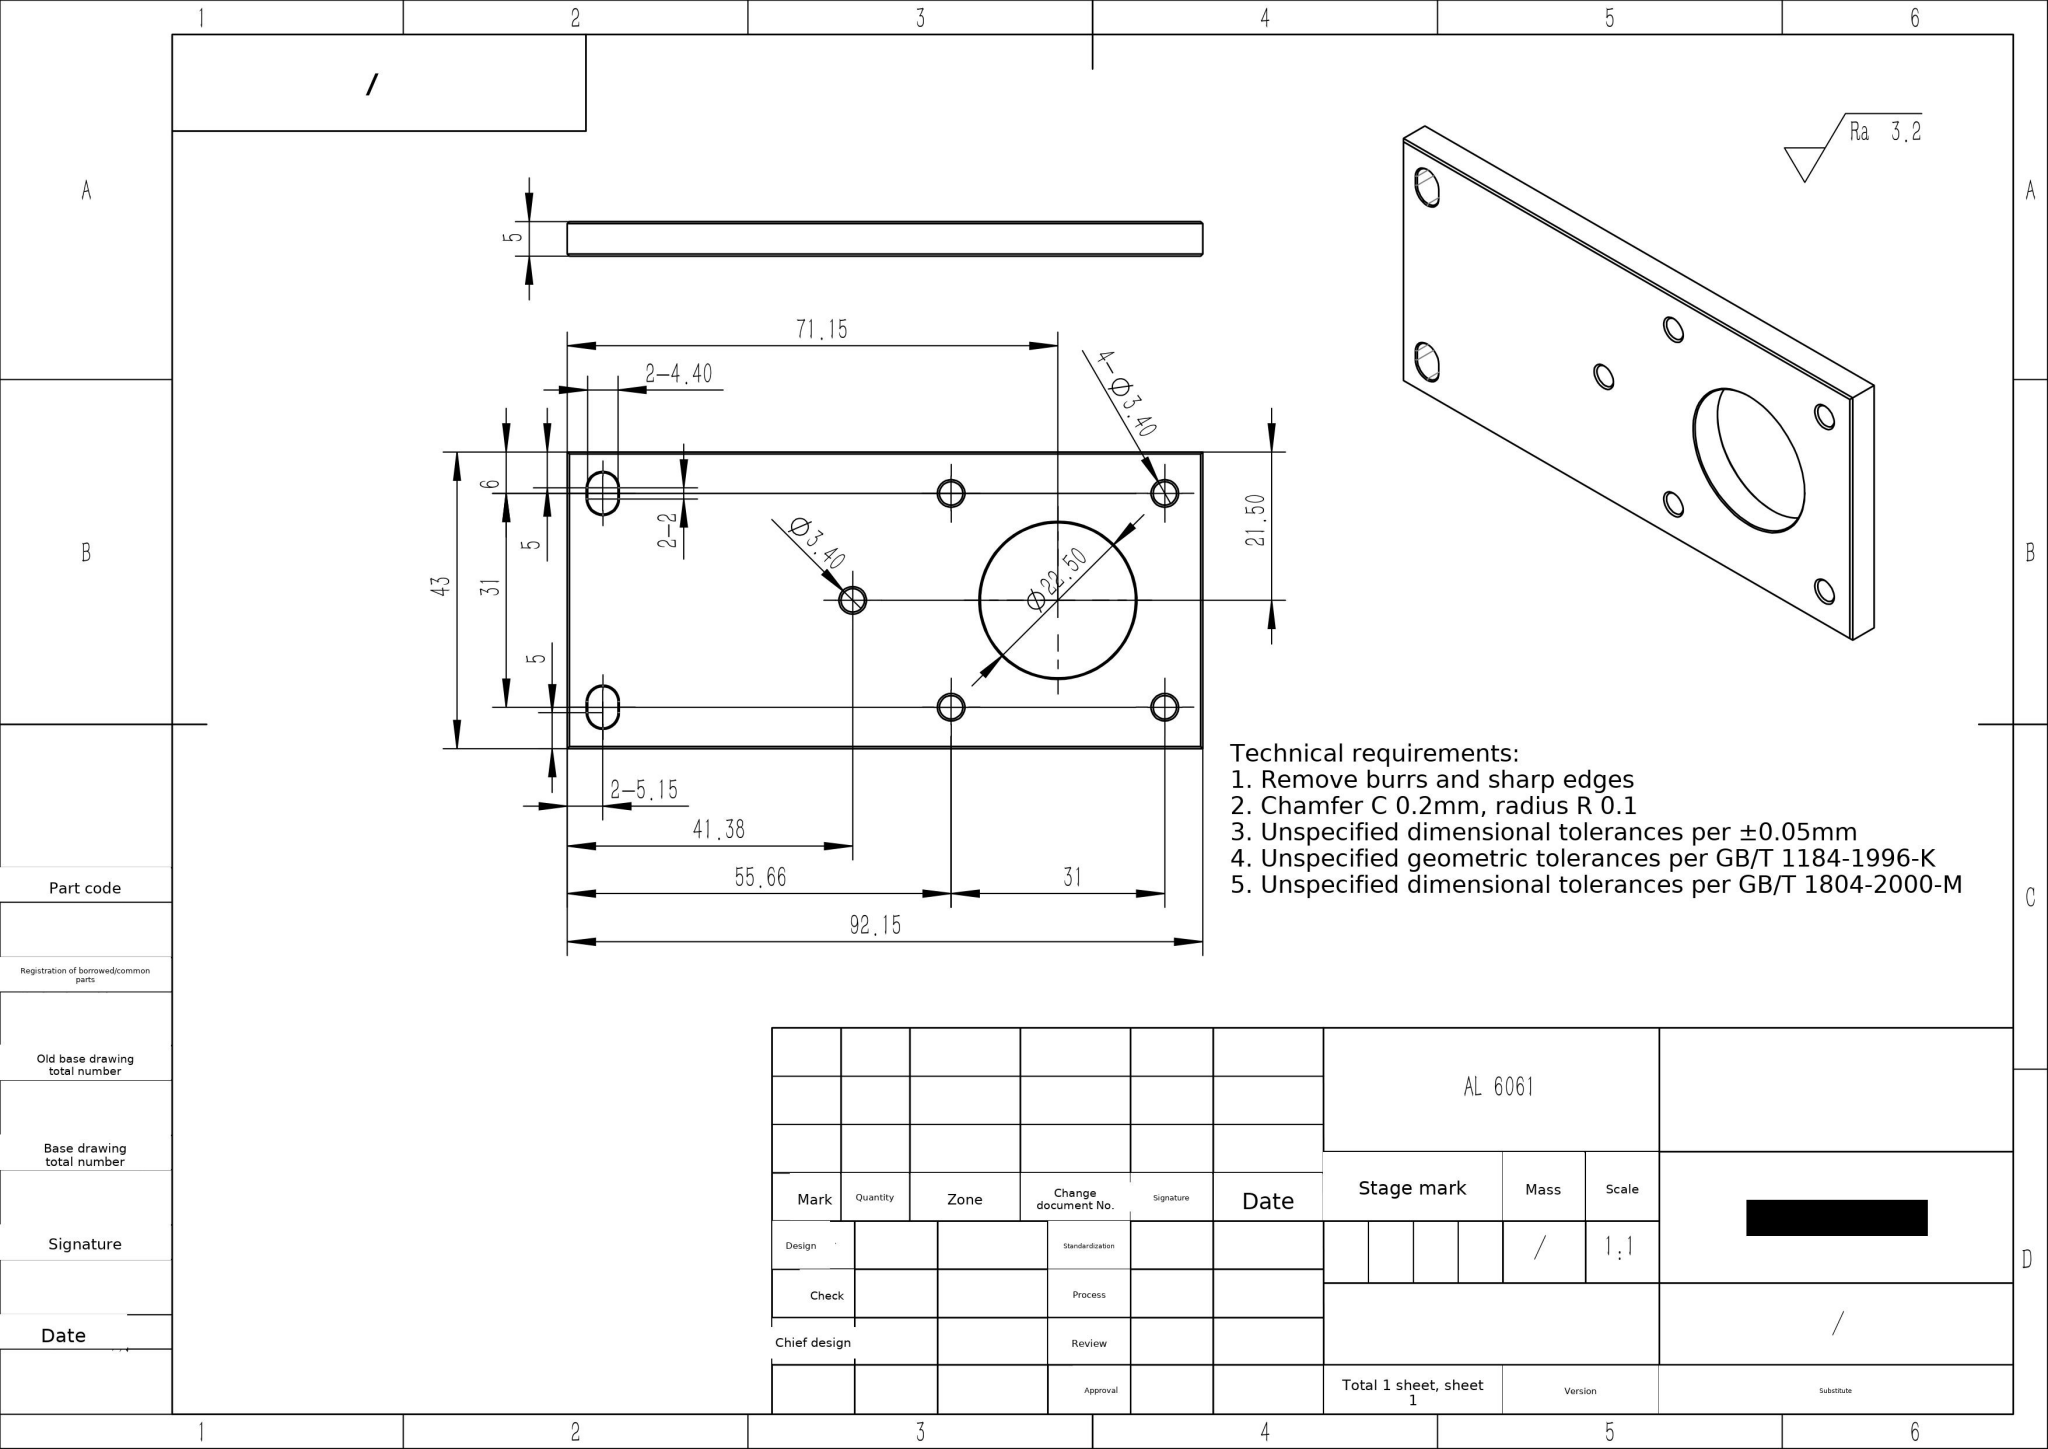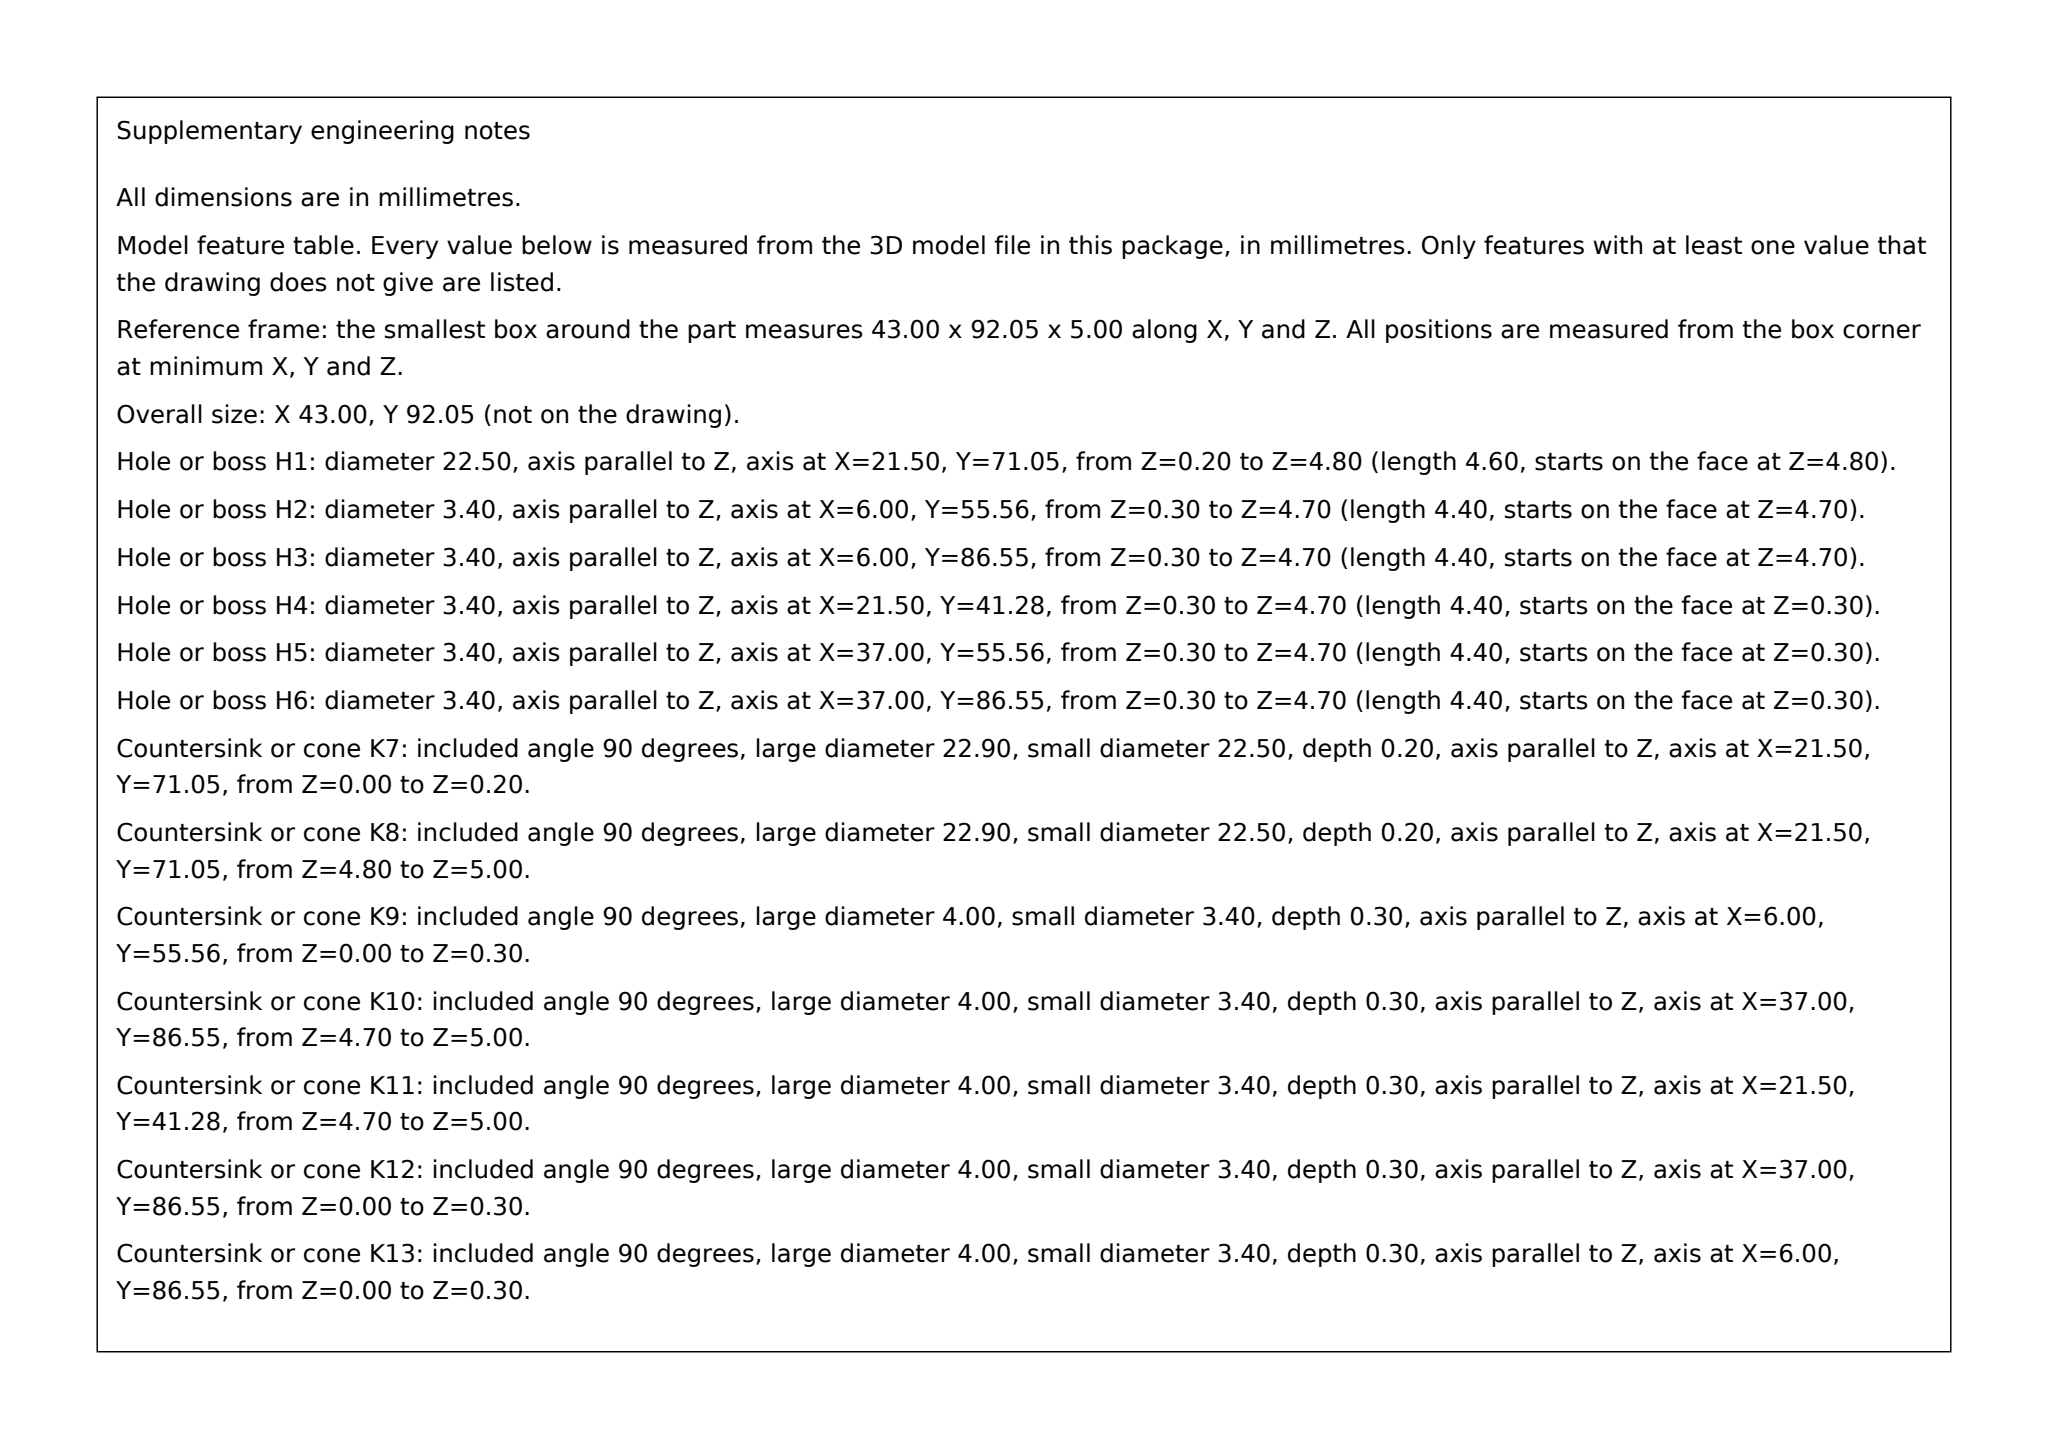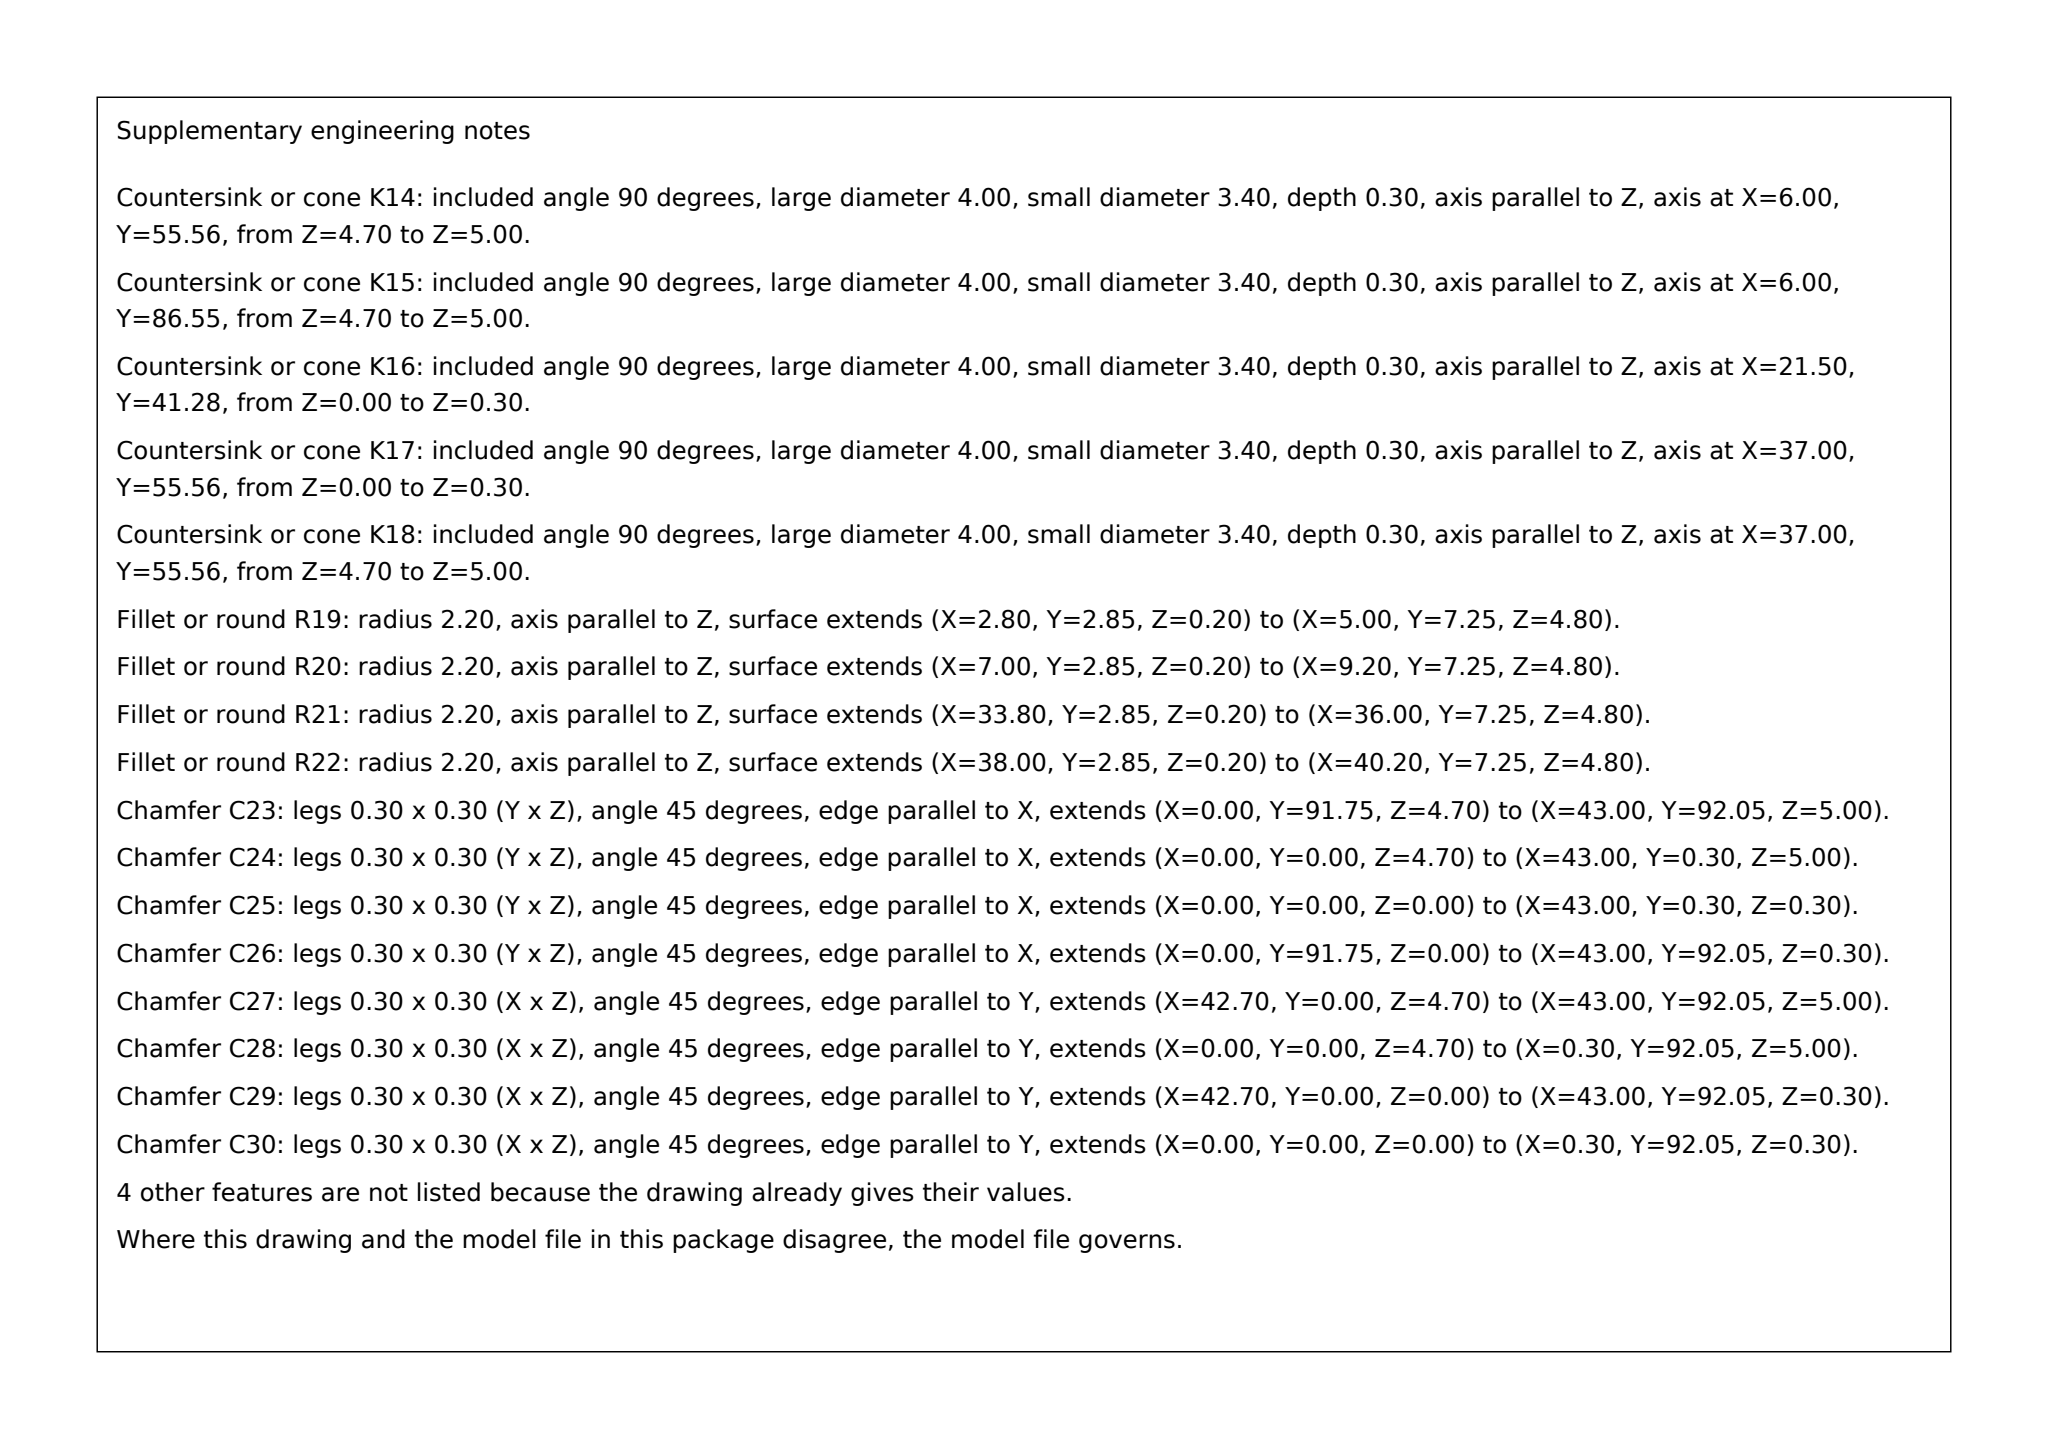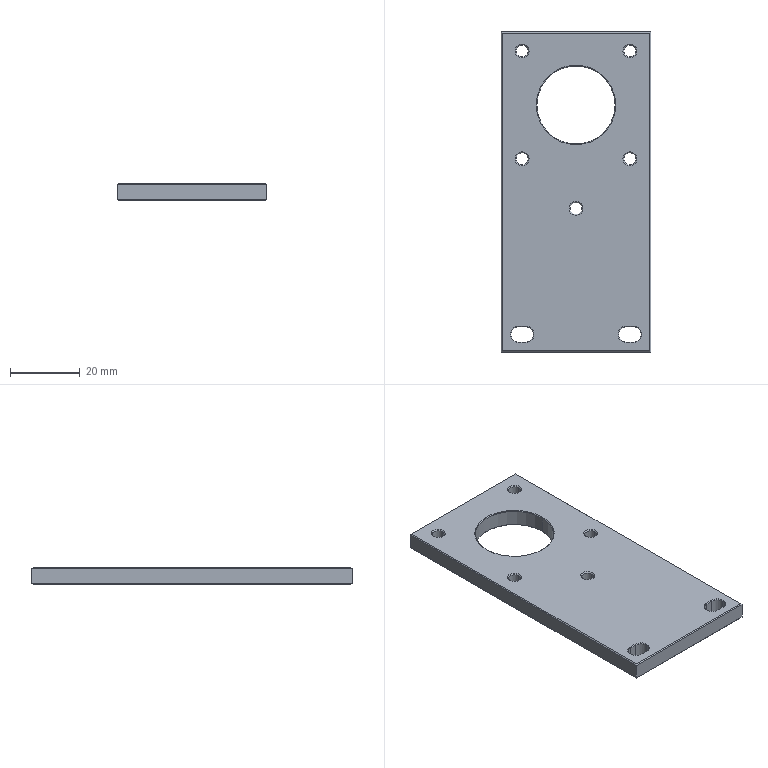Part | SolidWorks | mm | material AL 6061 | 1 solid | 86 faces | box 43 x 92.05 x 5 mm | volume 17302 mm3 | cone 40 | plane 26 | cylinder 20 | commonest cylinder face diameters 3.4 x10 4.4 x8 22.5 x2